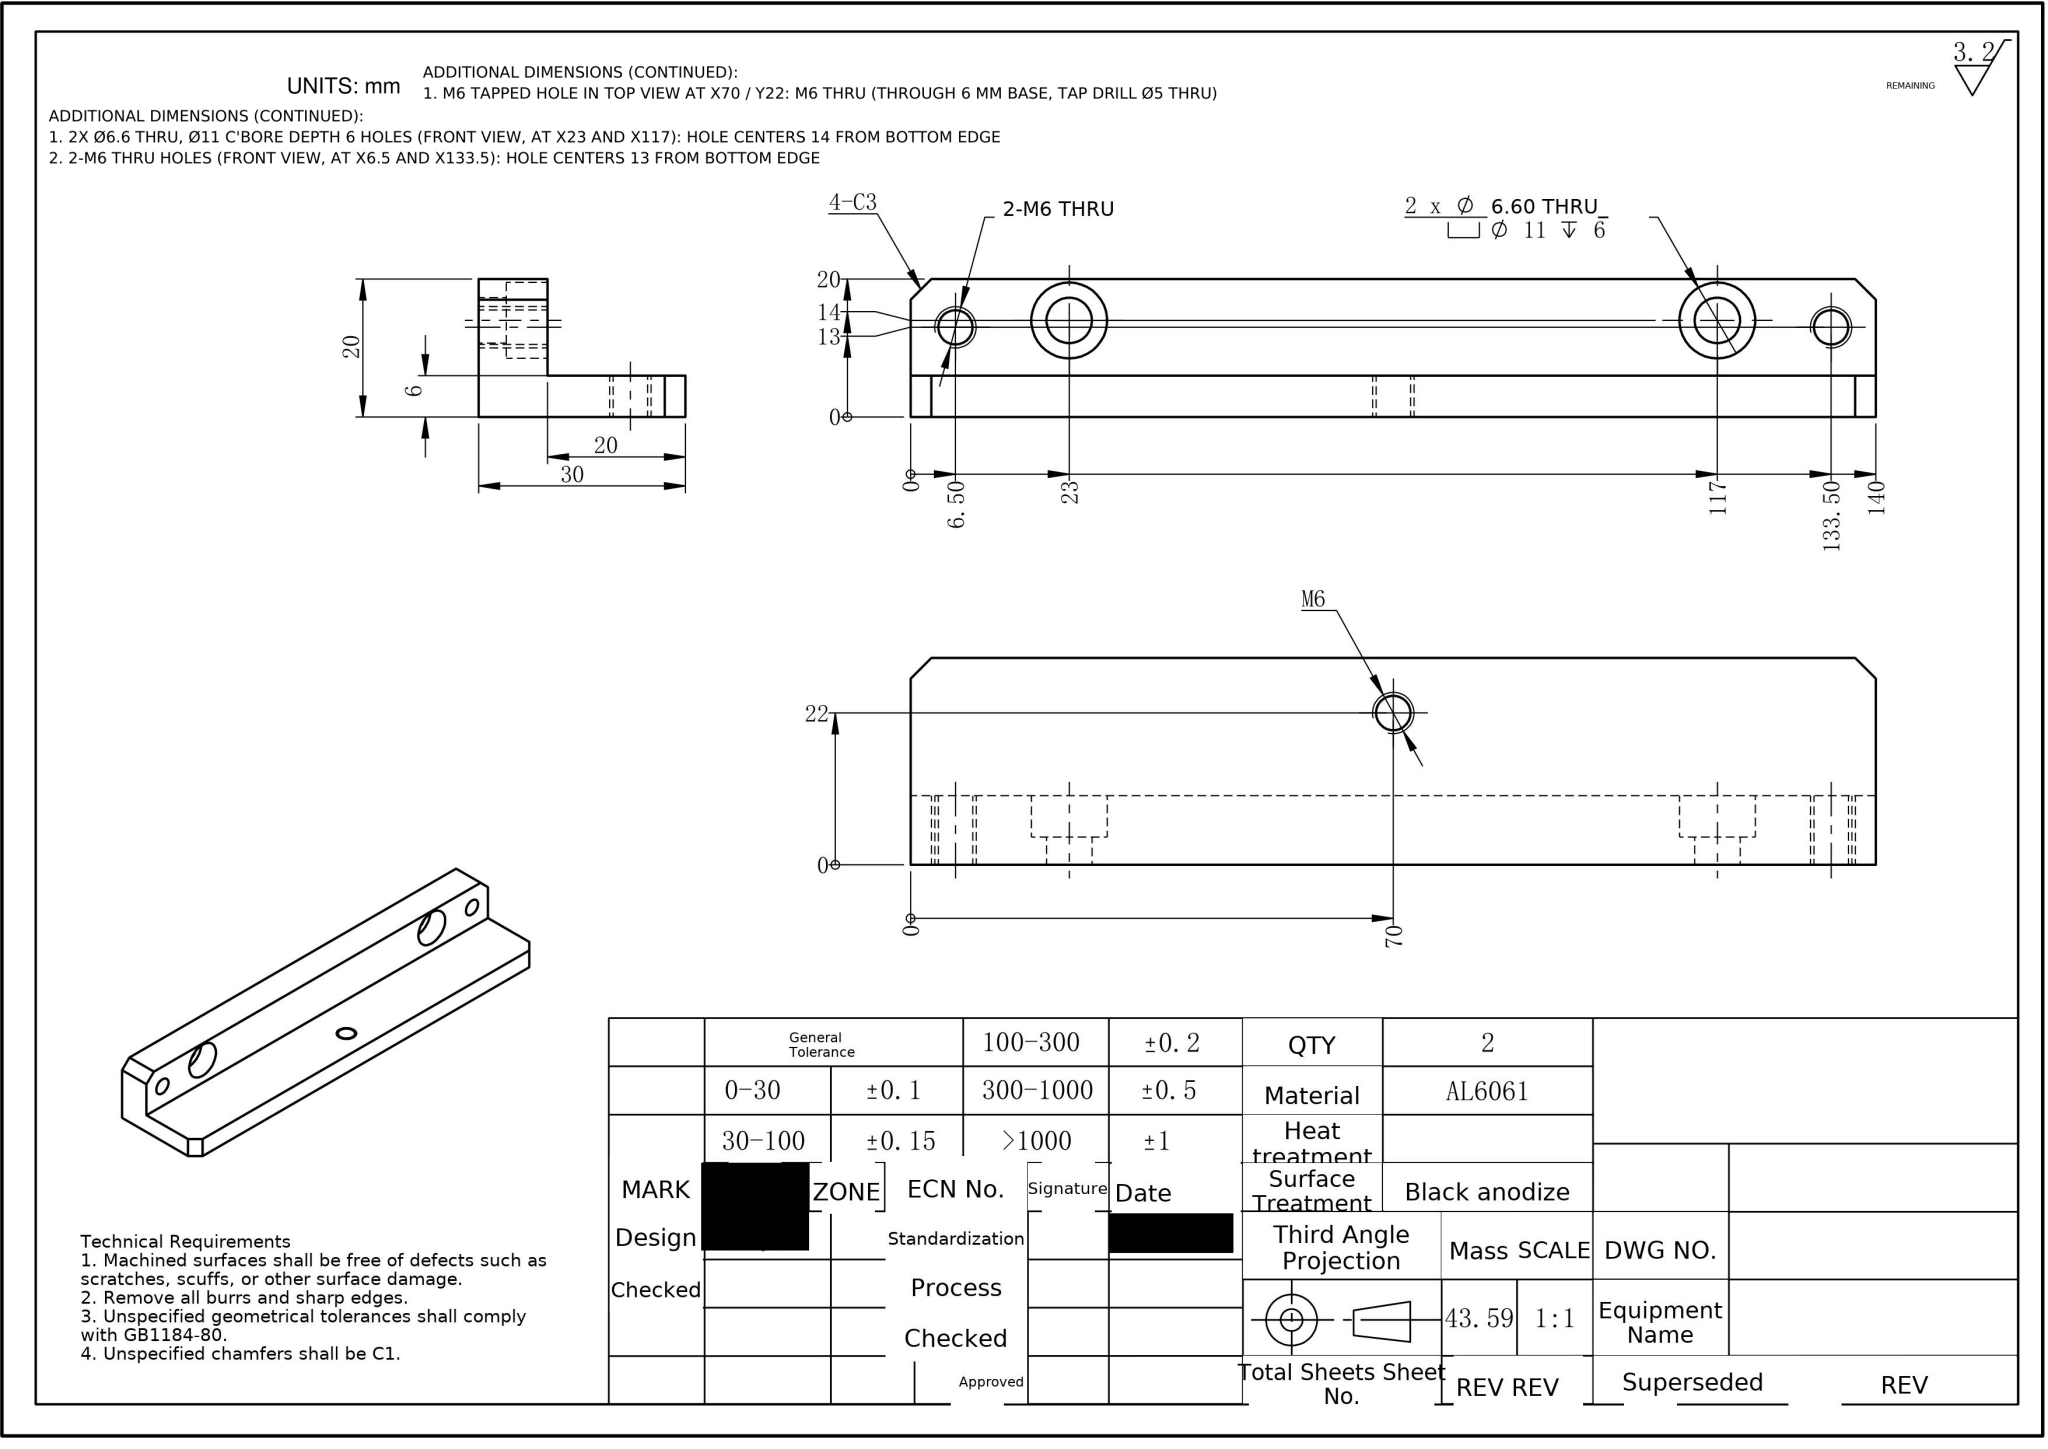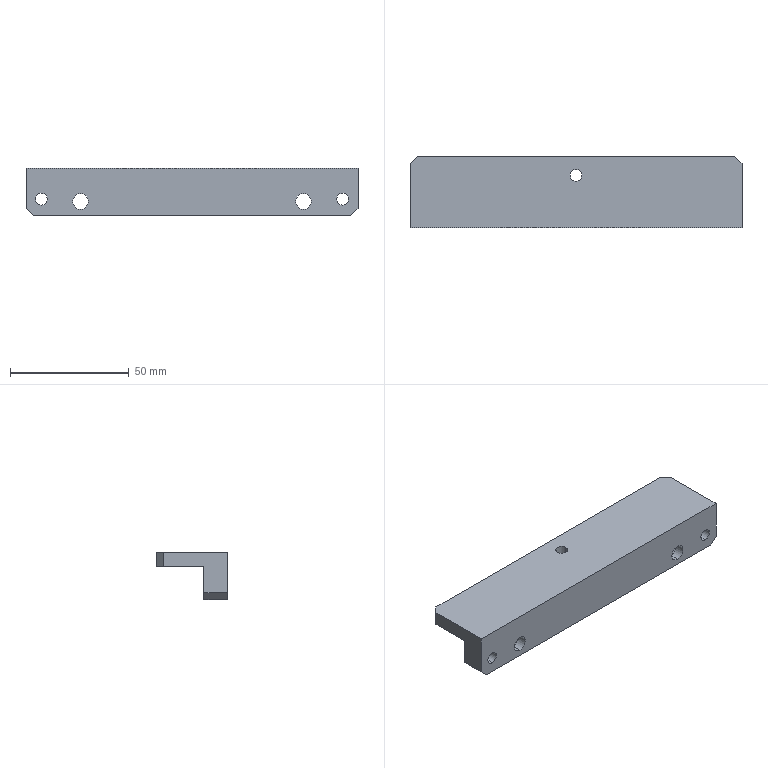Part | NX | mm | 1 solid | 28 faces | box 140 x 30 x 20 mm | volume 42731 mm3 | cylinder 14 | plane 14 | commonest cylinder face diameters 5 x6 11 x4 6.6 x4
STEP:
#1=COLOUR_RGB('',0.7922,0.8196,0.9333);
#2=FILL_AREA_STYLE_COLOUR('',#1);
#3=FILL_AREA_STYLE('',(#2));
#4=SURFACE_STYLE_FILL_AREA(#3);
#5=SURFACE_SIDE_STYLE('',(#4));
#6=SURFACE_STYLE_USAGE(.BOTH.,#5);
#7=PRESENTATION_STYLE_ASSIGNMENT((#6));
#8=CARTESIAN_POINT('',(2.5,17.,10.));
#9=VERTEX_POINT('',#8);
#10=CARTESIAN_POINT('',(-2.5,17.,10.));
#11=VERTEX_POINT('',#10);
#12=CARTESIAN_POINT('',(-0.,17.,10.));
#13=DIRECTION('',(0.,0.,-1.));
#14=DIRECTION('',(-1.,0.,0.));
#15=AXIS2_PLACEMENT_3D('',#12,#13,#14);
#16=CIRCLE('',#15,2.5);
#17=EDGE_CURVE('',#9,#11,#16,.T.);
#18=ORIENTED_EDGE('',*,*,#17,.F.);
#19=CARTESIAN_POINT('',(2.5,17.,4.));
#20=VERTEX_POINT('',#19);
#21=CARTESIAN_POINT('',(2.5,17.,4.));
#22=DIRECTION('',(0.,0.,-1.));
#23=VECTOR('',#22,1000.);
#24=LINE('',#21,#23);
#25=EDGE_CURVE('',#9,#20,#24,.T.);
#26=ORIENTED_EDGE('',*,*,#25,.T.);
#27=CARTESIAN_POINT('',(-2.5,17.,4.));
#28=VERTEX_POINT('',#27);
#29=CARTESIAN_POINT('',(-0.,17.,4.));
#30=DIRECTION('',(0.,0.,-1.));
#31=DIRECTION('',(-1.,0.,0.));
#32=AXIS2_PLACEMENT_3D('',#29,#30,#31);
#33=CIRCLE('',#32,2.5);
#34=EDGE_CURVE('',#20,#28,#33,.T.);
#35=ORIENTED_EDGE('',*,*,#34,.T.);
#36=CARTESIAN_POINT('',(-2.5,17.,4.));
#37=DIRECTION('',(0.,0.,-1.));
#38=VECTOR('',#37,1000.);
#39=LINE('',#36,#38);
#40=EDGE_CURVE('',#11,#28,#39,.T.);
#41=ORIENTED_EDGE('',*,*,#40,.F.);
#42=EDGE_LOOP('',(#18,#26,#35,#41));
#43=FACE_OUTER_BOUND('',#42,.T.);
#44=CARTESIAN_POINT('',(-0.,17.,4.));
#45=DIRECTION('',(0.,0.,-1.));
#46=DIRECTION('',(-1.,0.,0.));
#47=AXIS2_PLACEMENT_3D('',#44,#45,#46);
#48=CYLINDRICAL_SURFACE('',#47,2.5);
#49=ADVANCED_FACE('',(#43),#48,.F.);
#50=CARTESIAN_POINT('',(-63.5,5.,-0.5));
#51=VERTEX_POINT('',#50);
#52=CARTESIAN_POINT('',(-63.5,5.,-5.5));
#53=VERTEX_POINT('',#52);
#54=CARTESIAN_POINT('',(-63.5,5.,-3.));
#55=DIRECTION('',(0.,-1.,0.));
#56=DIRECTION('',(0.,0.,-1.));
#57=AXIS2_PLACEMENT_3D('',#54,#55,#56);
#58=CIRCLE('',#57,2.5);
#59=EDGE_CURVE('',#51,#53,#58,.T.);
#60=ORIENTED_EDGE('',*,*,#59,.F.);
#61=CARTESIAN_POINT('',(-63.5,-5.,-0.5));
#62=VERTEX_POINT('',#61);
#63=CARTESIAN_POINT('',(-63.5,-5.,-0.5));
#64=DIRECTION('',(0.,-1.,0.));
#65=VECTOR('',#64,1000.);
#66=LINE('',#63,#65);
#67=EDGE_CURVE('',#51,#62,#66,.T.);
#68=ORIENTED_EDGE('',*,*,#67,.T.);
#69=CARTESIAN_POINT('',(-63.5,-5.,-5.5));
#70=VERTEX_POINT('',#69);
#71=CARTESIAN_POINT('',(-63.5,-5.,-3.));
#72=DIRECTION('',(0.,-1.,0.));
#73=DIRECTION('',(0.,0.,-1.));
#74=AXIS2_PLACEMENT_3D('',#71,#72,#73);
#75=CIRCLE('',#74,2.5);
#76=EDGE_CURVE('',#62,#70,#75,.T.);
#77=ORIENTED_EDGE('',*,*,#76,.T.);
#78=CARTESIAN_POINT('',(-63.5,-5.,-5.5));
#79=DIRECTION('',(0.,-1.,0.));
#80=VECTOR('',#79,1000.);
#81=LINE('',#78,#80);
#82=EDGE_CURVE('',#53,#70,#81,.T.);
#83=ORIENTED_EDGE('',*,*,#82,.F.);
#84=EDGE_LOOP('',(#60,#68,#77,#83));
#85=FACE_OUTER_BOUND('',#84,.T.);
#86=CARTESIAN_POINT('',(-63.5,-5.,-3.));
#87=DIRECTION('',(0.,-1.,0.));
#88=DIRECTION('',(0.,0.,-1.));
#89=AXIS2_PLACEMENT_3D('',#86,#87,#88);
#90=CYLINDRICAL_SURFACE('',#89,2.5);
#91=ADVANCED_FACE('',(#85),#90,.F.);
#92=CARTESIAN_POINT('',(63.5,5.,-0.5));
#93=VERTEX_POINT('',#92);
#94=CARTESIAN_POINT('',(63.5,5.,-5.5));
#95=VERTEX_POINT('',#94);
#96=CARTESIAN_POINT('',(63.5,5.,-3.));
#97=DIRECTION('',(0.,-1.,0.));
#98=DIRECTION('',(0.,0.,-1.));
#99=AXIS2_PLACEMENT_3D('',#96,#97,#98);
#100=CIRCLE('',#99,2.5);
#101=EDGE_CURVE('',#93,#95,#100,.T.);
#102=ORIENTED_EDGE('',*,*,#101,.F.);
#103=CARTESIAN_POINT('',(63.5,-5.,-0.5));
#104=VERTEX_POINT('',#103);
#105=CARTESIAN_POINT('',(63.5,-5.,-0.5));
#106=DIRECTION('',(0.,-1.,0.));
#107=VECTOR('',#106,1000.);
#108=LINE('',#105,#107);
#109=EDGE_CURVE('',#93,#104,#108,.T.);
#110=ORIENTED_EDGE('',*,*,#109,.T.);
#111=CARTESIAN_POINT('',(63.5,-5.,-5.5));
#112=VERTEX_POINT('',#111);
#113=CARTESIAN_POINT('',(63.5,-5.,-3.));
#114=DIRECTION('',(0.,-1.,0.));
#115=DIRECTION('',(0.,0.,-1.));
#116=AXIS2_PLACEMENT_3D('',#113,#114,#115);
#117=CIRCLE('',#116,2.5);
#118=EDGE_CURVE('',#104,#112,#117,.T.);
#119=ORIENTED_EDGE('',*,*,#118,.T.);
#120=CARTESIAN_POINT('',(63.5,-5.,-5.5));
#121=DIRECTION('',(0.,-1.,0.));
#122=VECTOR('',#121,1000.);
#123=LINE('',#120,#122);
#124=EDGE_CURVE('',#95,#112,#123,.T.);
#125=ORIENTED_EDGE('',*,*,#124,.F.);
#126=EDGE_LOOP('',(#102,#110,#119,#125));
#127=FACE_OUTER_BOUND('',#126,.T.);
#128=CARTESIAN_POINT('',(63.5,-5.,-3.));
#129=DIRECTION('',(0.,-1.,0.));
#130=DIRECTION('',(0.,0.,-1.));
#131=AXIS2_PLACEMENT_3D('',#128,#129,#130);
#132=CYLINDRICAL_SURFACE('',#131,2.5);
#133=ADVANCED_FACE('',(#127),#132,.F.);
#134=CARTESIAN_POINT('',(-47.,-1.,-9.5));
#135=VERTEX_POINT('',#134);
#136=CARTESIAN_POINT('',(-47.,-1.,1.5));
#137=VERTEX_POINT('',#136);
#138=CARTESIAN_POINT('',(-47.,-1.,-4.));
#139=DIRECTION('',(0.,1.,0.));
#140=DIRECTION('',(0.,0.,1.));
#141=AXIS2_PLACEMENT_3D('',#138,#139,#140);
#142=CIRCLE('',#141,5.5);
#143=EDGE_CURVE('',#135,#137,#142,.T.);
#144=ORIENTED_EDGE('',*,*,#143,.F.);
#145=CARTESIAN_POINT('',(-47.,5.,-9.5));
#146=VERTEX_POINT('',#145);
#147=CARTESIAN_POINT('',(-47.,5.,-9.5));
#148=DIRECTION('',(0.,1.,0.));
#149=VECTOR('',#148,1000.);
#150=LINE('',#147,#149);
#151=EDGE_CURVE('',#135,#146,#150,.T.);
#152=ORIENTED_EDGE('',*,*,#151,.T.);
#153=CARTESIAN_POINT('',(-47.,5.,1.5));
#154=VERTEX_POINT('',#153);
#155=CARTESIAN_POINT('',(-47.,5.,-4.));
#156=DIRECTION('',(0.,1.,0.));
#157=DIRECTION('',(0.,0.,1.));
#158=AXIS2_PLACEMENT_3D('',#155,#156,#157);
#159=CIRCLE('',#158,5.5);
#160=EDGE_CURVE('',#146,#154,#159,.T.);
#161=ORIENTED_EDGE('',*,*,#160,.T.);
#162=CARTESIAN_POINT('',(-47.,5.,1.5));
#163=DIRECTION('',(0.,1.,0.));
#164=VECTOR('',#163,1000.);
#165=LINE('',#162,#164);
#166=EDGE_CURVE('',#137,#154,#165,.T.);
#167=ORIENTED_EDGE('',*,*,#166,.F.);
#168=EDGE_LOOP('',(#144,#152,#161,#167));
#169=FACE_OUTER_BOUND('',#168,.T.);
#170=CARTESIAN_POINT('',(-47.,5.,-4.));
#171=DIRECTION('',(0.,1.,0.));
#172=DIRECTION('',(0.,0.,1.));
#173=AXIS2_PLACEMENT_3D('',#170,#171,#172);
#174=CYLINDRICAL_SURFACE('',#173,5.5);
#175=ADVANCED_FACE('',(#169),#174,.F.);
#176=CARTESIAN_POINT('',(-47.,-5.,-7.3));
#177=VERTEX_POINT('',#176);
#178=CARTESIAN_POINT('',(-47.,-5.,-0.7));
#179=VERTEX_POINT('',#178);
#180=CARTESIAN_POINT('',(-47.,-5.,-4.));
#181=DIRECTION('',(0.,1.,0.));
#182=DIRECTION('',(0.,0.,1.));
#183=AXIS2_PLACEMENT_3D('',#180,#181,#182);
#184=CIRCLE('',#183,3.3);
#185=EDGE_CURVE('',#177,#179,#184,.T.);
#186=ORIENTED_EDGE('',*,*,#185,.F.);
#187=CARTESIAN_POINT('',(-47.,-1.,-7.3));
#188=VERTEX_POINT('',#187);
#189=CARTESIAN_POINT('',(-47.,5.,-7.3));
#190=DIRECTION('',(0.,1.,0.));
#191=VECTOR('',#190,1000.);
#192=LINE('',#189,#191);
#193=EDGE_CURVE('',#177,#188,#192,.T.);
#194=ORIENTED_EDGE('',*,*,#193,.T.);
#195=CARTESIAN_POINT('',(-47.,-1.,-0.7));
#196=VERTEX_POINT('',#195);
#197=CARTESIAN_POINT('',(-47.,-1.,-4.));
#198=DIRECTION('',(0.,1.,0.));
#199=DIRECTION('',(0.,0.,1.));
#200=AXIS2_PLACEMENT_3D('',#197,#198,#199);
#201=CIRCLE('',#200,3.3);
#202=EDGE_CURVE('',#188,#196,#201,.T.);
#203=ORIENTED_EDGE('',*,*,#202,.T.);
#204=CARTESIAN_POINT('',(-47.,5.,-0.7));
#205=DIRECTION('',(0.,1.,0.));
#206=VECTOR('',#205,1000.);
#207=LINE('',#204,#206);
#208=EDGE_CURVE('',#179,#196,#207,.T.);
#209=ORIENTED_EDGE('',*,*,#208,.F.);
#210=EDGE_LOOP('',(#186,#194,#203,#209));
#211=FACE_OUTER_BOUND('',#210,.T.);
#212=CARTESIAN_POINT('',(-47.,5.,-4.));
#213=DIRECTION('',(0.,1.,0.));
#214=DIRECTION('',(0.,0.,1.));
#215=AXIS2_PLACEMENT_3D('',#212,#213,#214);
#216=CYLINDRICAL_SURFACE('',#215,3.3);
#217=ADVANCED_FACE('',(#211),#216,.F.);
#218=CARTESIAN_POINT('',(47.,-1.,-9.5));
#219=VERTEX_POINT('',#218);
#220=CARTESIAN_POINT('',(47.,-1.,1.5));
#221=VERTEX_POINT('',#220);
#222=CARTESIAN_POINT('',(47.,-1.,-4.));
#223=DIRECTION('',(0.,1.,0.));
#224=DIRECTION('',(0.,0.,1.));
#225=AXIS2_PLACEMENT_3D('',#222,#223,#224);
#226=CIRCLE('',#225,5.5);
#227=EDGE_CURVE('',#219,#221,#226,.T.);
#228=ORIENTED_EDGE('',*,*,#227,.F.);
#229=CARTESIAN_POINT('',(47.,5.,-9.5));
#230=VERTEX_POINT('',#229);
#231=CARTESIAN_POINT('',(47.,5.,-9.5));
#232=DIRECTION('',(0.,1.,0.));
#233=VECTOR('',#232,1000.);
#234=LINE('',#231,#233);
#235=EDGE_CURVE('',#219,#230,#234,.T.);
#236=ORIENTED_EDGE('',*,*,#235,.T.);
#237=CARTESIAN_POINT('',(47.,5.,1.5));
#238=VERTEX_POINT('',#237);
#239=CARTESIAN_POINT('',(47.,5.,-4.));
#240=DIRECTION('',(0.,1.,0.));
#241=DIRECTION('',(0.,0.,1.));
#242=AXIS2_PLACEMENT_3D('',#239,#240,#241);
#243=CIRCLE('',#242,5.5);
#244=EDGE_CURVE('',#230,#238,#243,.T.);
#245=ORIENTED_EDGE('',*,*,#244,.T.);
#246=CARTESIAN_POINT('',(47.,5.,1.5));
#247=DIRECTION('',(0.,1.,0.));
#248=VECTOR('',#247,1000.);
#249=LINE('',#246,#248);
#250=EDGE_CURVE('',#221,#238,#249,.T.);
#251=ORIENTED_EDGE('',*,*,#250,.F.);
#252=EDGE_LOOP('',(#228,#236,#245,#251));
#253=FACE_OUTER_BOUND('',#252,.T.);
#254=CARTESIAN_POINT('',(47.,5.,-4.));
#255=DIRECTION('',(0.,1.,0.));
#256=DIRECTION('',(0.,0.,1.));
#257=AXIS2_PLACEMENT_3D('',#254,#255,#256);
#258=CYLINDRICAL_SURFACE('',#257,5.5);
#259=ADVANCED_FACE('',(#253),#258,.F.);
#260=CARTESIAN_POINT('',(47.,-5.,-7.3));
#261=VERTEX_POINT('',#260);
#262=CARTESIAN_POINT('',(47.,-5.,-0.7));
#263=VERTEX_POINT('',#262);
#264=CARTESIAN_POINT('',(47.,-5.,-4.));
#265=DIRECTION('',(0.,1.,0.));
#266=DIRECTION('',(0.,0.,1.));
#267=AXIS2_PLACEMENT_3D('',#264,#265,#266);
#268=CIRCLE('',#267,3.3);
#269=EDGE_CURVE('',#261,#263,#268,.T.);
#270=ORIENTED_EDGE('',*,*,#269,.F.);
#271=CARTESIAN_POINT('',(47.,-1.,-7.3));
#272=VERTEX_POINT('',#271);
#273=CARTESIAN_POINT('',(47.,5.,-7.3));
#274=DIRECTION('',(0.,1.,0.));
#275=VECTOR('',#274,1000.);
#276=LINE('',#273,#275);
#277=EDGE_CURVE('',#261,#272,#276,.T.);
#278=ORIENTED_EDGE('',*,*,#277,.T.);
#279=CARTESIAN_POINT('',(47.,-1.,-0.7));
#280=VERTEX_POINT('',#279);
#281=CARTESIAN_POINT('',(47.,-1.,-4.));
#282=DIRECTION('',(0.,1.,0.));
#283=DIRECTION('',(0.,0.,1.));
#284=AXIS2_PLACEMENT_3D('',#281,#282,#283);
#285=CIRCLE('',#284,3.3);
#286=EDGE_CURVE('',#272,#280,#285,.T.);
#287=ORIENTED_EDGE('',*,*,#286,.T.);
#288=CARTESIAN_POINT('',(47.,5.,-0.7));
#289=DIRECTION('',(0.,1.,0.));
#290=VECTOR('',#289,1000.);
#291=LINE('',#288,#290);
#292=EDGE_CURVE('',#263,#280,#291,.T.);
#293=ORIENTED_EDGE('',*,*,#292,.F.);
#294=EDGE_LOOP('',(#270,#278,#287,#293));
#295=FACE_OUTER_BOUND('',#294,.T.);
#296=CARTESIAN_POINT('',(47.,5.,-4.));
#297=DIRECTION('',(0.,1.,0.));
#298=DIRECTION('',(0.,0.,1.));
#299=AXIS2_PLACEMENT_3D('',#296,#297,#298);
#300=CYLINDRICAL_SURFACE('',#299,3.3);
#301=ADVANCED_FACE('',(#295),#300,.F.);
#302=CARTESIAN_POINT('',(-63.5,5.,-3.));
#303=DIRECTION('',(0.,-1.,0.));
#304=DIRECTION('',(0.,0.,-1.));
#305=AXIS2_PLACEMENT_3D('',#302,#303,#304);
#306=CIRCLE('',#305,2.5);
#307=EDGE_CURVE('',#53,#51,#306,.T.);
#308=ORIENTED_EDGE('',*,*,#307,.T.);
#309=ORIENTED_EDGE('',*,*,#59,.T.);
#310=EDGE_LOOP('',(#308,#309));
#311=FACE_BOUND('',#310,.T.);
#312=CARTESIAN_POINT('',(63.5,5.,-3.));
#313=DIRECTION('',(0.,-1.,0.));
#314=DIRECTION('',(0.,0.,-1.));
#315=AXIS2_PLACEMENT_3D('',#312,#313,#314);
#316=CIRCLE('',#315,2.5);
#317=EDGE_CURVE('',#95,#93,#316,.T.);
#318=ORIENTED_EDGE('',*,*,#317,.T.);
#319=ORIENTED_EDGE('',*,*,#101,.T.);
#320=EDGE_LOOP('',(#318,#319));
#321=FACE_BOUND('',#320,.T.);
#322=CARTESIAN_POINT('',(47.,5.,-4.));
#323=DIRECTION('',(0.,1.,0.));
#324=DIRECTION('',(0.,0.,1.));
#325=AXIS2_PLACEMENT_3D('',#322,#323,#324);
#326=CIRCLE('',#325,5.5);
#327=EDGE_CURVE('',#238,#230,#326,.T.);
#328=ORIENTED_EDGE('',*,*,#327,.F.);
#329=ORIENTED_EDGE('',*,*,#244,.F.);
#330=EDGE_LOOP('',(#328,#329));
#331=FACE_BOUND('',#330,.T.);
#332=CARTESIAN_POINT('',(-47.,5.,-4.));
#333=DIRECTION('',(0.,1.,0.));
#334=DIRECTION('',(0.,0.,1.));
#335=AXIS2_PLACEMENT_3D('',#332,#333,#334);
#336=CIRCLE('',#335,5.5);
#337=EDGE_CURVE('',#154,#146,#336,.T.);
#338=ORIENTED_EDGE('',*,*,#337,.F.);
#339=ORIENTED_EDGE('',*,*,#160,.F.);
#340=EDGE_LOOP('',(#338,#339));
#341=FACE_BOUND('',#340,.T.);
#342=CARTESIAN_POINT('',(70.,5.,4.));
#343=VERTEX_POINT('',#342);
#344=CARTESIAN_POINT('',(70.,5.,-7.));
#345=VERTEX_POINT('',#344);
#346=CARTESIAN_POINT('',(70.,5.,10.));
#347=DIRECTION('',(0.,0.,-1.));
#348=VECTOR('',#347,1000.);
#349=LINE('',#346,#348);
#350=EDGE_CURVE('',#343,#345,#349,.T.);
#351=ORIENTED_EDGE('',*,*,#350,.T.);
#352=CARTESIAN_POINT('',(67.,5.,-10.));
#353=VERTEX_POINT('',#352);
#354=CARTESIAN_POINT('',(67.,5.,-10.));
#355=DIRECTION('',(-0.7071,0.,-0.7071));
#356=VECTOR('',#355,1000.);
#357=LINE('',#354,#356);
#358=EDGE_CURVE('',#345,#353,#357,.T.);
#359=ORIENTED_EDGE('',*,*,#358,.T.);
#360=CARTESIAN_POINT('',(-67.,5.,-10.));
#361=VERTEX_POINT('',#360);
#362=CARTESIAN_POINT('',(-70.,5.,-10.));
#363=DIRECTION('',(-1.,0.,0.));
#364=VECTOR('',#363,1000.);
#365=LINE('',#362,#364);
#366=EDGE_CURVE('',#353,#361,#365,.T.);
#367=ORIENTED_EDGE('',*,*,#366,.T.);
#368=CARTESIAN_POINT('',(-70.,5.,-7.));
#369=VERTEX_POINT('',#368);
#370=CARTESIAN_POINT('',(-70.,5.,-7.));
#371=DIRECTION('',(-0.7071,0.,0.7071));
#372=VECTOR('',#371,1000.);
#373=LINE('',#370,#372);
#374=EDGE_CURVE('',#361,#369,#373,.T.);
#375=ORIENTED_EDGE('',*,*,#374,.T.);
#376=CARTESIAN_POINT('',(-70.,5.,4.));
#377=VERTEX_POINT('',#376);
#378=CARTESIAN_POINT('',(-70.,5.,10.));
#379=DIRECTION('',(0.,0.,1.));
#380=VECTOR('',#379,1000.);
#381=LINE('',#378,#380);
#382=EDGE_CURVE('',#369,#377,#381,.T.);
#383=ORIENTED_EDGE('',*,*,#382,.T.);
#384=CARTESIAN_POINT('',(-70.,5.,4.));
#385=DIRECTION('',(-1.,0.,0.));
#386=VECTOR('',#385,1000.);
#387=LINE('',#384,#386);
#388=EDGE_CURVE('',#343,#377,#387,.T.);
#389=ORIENTED_EDGE('',*,*,#388,.F.);
#390=EDGE_LOOP('',(#351,#359,#367,#375,#383,#389));
#391=FACE_OUTER_BOUND('',#390,.T.);
#392=CARTESIAN_POINT('',(0.,5.,0.));
#393=DIRECTION('',(0.,-1.,0.));
#394=DIRECTION('',(0.,0.,-1.));
#395=AXIS2_PLACEMENT_3D('',#392,#393,#394);
#396=PLANE('',#395);
#397=ADVANCED_FACE('',(#311,#321,#331,#341,#391),#396,.F.);
#398=CARTESIAN_POINT('',(70.,-5.,10.));
#399=VERTEX_POINT('',#398);
#400=CARTESIAN_POINT('',(70.,-5.,-7.));
#401=VERTEX_POINT('',#400);
#402=CARTESIAN_POINT('',(70.,-5.,10.));
#403=DIRECTION('',(0.,0.,-1.));
#404=VECTOR('',#403,1000.);
#405=LINE('',#402,#404);
#406=EDGE_CURVE('',#399,#401,#405,.T.);
#407=ORIENTED_EDGE('',*,*,#406,.T.);
#408=CARTESIAN_POINT('',(70.,5.,-7.));
#409=DIRECTION('',(0.,1.,0.));
#410=VECTOR('',#409,1000.);
#411=LINE('',#408,#410);
#412=EDGE_CURVE('',#401,#345,#411,.T.);
#413=ORIENTED_EDGE('',*,*,#412,.T.);
#414=ORIENTED_EDGE('',*,*,#350,.F.);
#415=CARTESIAN_POINT('',(70.,22.,4.));
#416=VERTEX_POINT('',#415);
#417=CARTESIAN_POINT('',(70.,25.,4.));
#418=DIRECTION('',(0.,-1.,0.));
#419=VECTOR('',#418,1000.);
#420=LINE('',#417,#419);
#421=EDGE_CURVE('',#416,#343,#420,.T.);
#422=ORIENTED_EDGE('',*,*,#421,.F.);
#423=CARTESIAN_POINT('',(70.,22.,10.));
#424=VERTEX_POINT('',#423);
#425=CARTESIAN_POINT('',(70.,22.,10.));
#426=DIRECTION('',(0.,0.,1.));
#427=VECTOR('',#426,1000.);
#428=LINE('',#425,#427);
#429=EDGE_CURVE('',#416,#424,#428,.T.);
#430=ORIENTED_EDGE('',*,*,#429,.T.);
#431=CARTESIAN_POINT('',(70.,5.,10.));
#432=DIRECTION('',(0.,-1.,0.));
#433=VECTOR('',#432,1000.);
#434=LINE('',#431,#433);
#435=EDGE_CURVE('',#424,#399,#434,.T.);
#436=ORIENTED_EDGE('',*,*,#435,.T.);
#437=EDGE_LOOP('',(#407,#413,#414,#422,#430,#436));
#438=FACE_OUTER_BOUND('',#437,.T.);
#439=CARTESIAN_POINT('',(70.,5.,10.));
#440=DIRECTION('',(-1.,0.,0.));
#441=DIRECTION('',(0.,0.,1.));
#442=AXIS2_PLACEMENT_3D('',#439,#440,#441);
#443=PLANE('',#442);
#444=ADVANCED_FACE('',(#438),#443,.F.);
#445=ORIENTED_EDGE('',*,*,#366,.F.);
#446=CARTESIAN_POINT('',(67.,-5.,-10.));
#447=VERTEX_POINT('',#446);
#448=CARTESIAN_POINT('',(67.,5.,-10.));
#449=DIRECTION('',(0.,-1.,0.));
#450=VECTOR('',#449,1000.);
#451=LINE('',#448,#450);
#452=EDGE_CURVE('',#353,#447,#451,.T.);
#453=ORIENTED_EDGE('',*,*,#452,.T.);
#454=CARTESIAN_POINT('',(-67.,-5.,-10.));
#455=VERTEX_POINT('',#454);
#456=CARTESIAN_POINT('',(-70.,-5.,-10.));
#457=DIRECTION('',(-1.,0.,0.));
#458=VECTOR('',#457,1000.);
#459=LINE('',#456,#458);
#460=EDGE_CURVE('',#447,#455,#459,.T.);
#461=ORIENTED_EDGE('',*,*,#460,.T.);
#462=CARTESIAN_POINT('',(-67.,5.,-10.));
#463=DIRECTION('',(0.,1.,0.));
#464=VECTOR('',#463,1000.);
#465=LINE('',#462,#464);
#466=EDGE_CURVE('',#455,#361,#465,.T.);
#467=ORIENTED_EDGE('',*,*,#466,.T.);
#468=EDGE_LOOP('',(#445,#453,#461,#467));
#469=FACE_OUTER_BOUND('',#468,.T.);
#470=CARTESIAN_POINT('',(-70.,5.,-10.));
#471=DIRECTION('',(0.,0.,1.));
#472=DIRECTION('',(1.,0.,0.));
#473=AXIS2_PLACEMENT_3D('',#470,#471,#472);
#474=PLANE('',#473);
#475=ADVANCED_FACE('',(#469),#474,.F.);
#476=ORIENTED_EDGE('',*,*,#382,.F.);
#477=CARTESIAN_POINT('',(-70.,-5.,-7.));
#478=VERTEX_POINT('',#477);
#479=CARTESIAN_POINT('',(-70.,5.,-7.));
#480=DIRECTION('',(0.,-1.,0.));
#481=VECTOR('',#480,1000.);
#482=LINE('',#479,#481);
#483=EDGE_CURVE('',#369,#478,#482,.T.);
#484=ORIENTED_EDGE('',*,*,#483,.T.);
#485=CARTESIAN_POINT('',(-70.,-5.,10.));
#486=VERTEX_POINT('',#485);
#487=CARTESIAN_POINT('',(-70.,-5.,10.));
#488=DIRECTION('',(0.,0.,1.));
#489=VECTOR('',#488,1000.);
#490=LINE('',#487,#489);
#491=EDGE_CURVE('',#478,#486,#490,.T.);
#492=ORIENTED_EDGE('',*,*,#491,.T.);
#493=CARTESIAN_POINT('',(-70.,22.,10.));
#494=VERTEX_POINT('',#493);
#495=CARTESIAN_POINT('',(-70.,5.,10.));
#496=DIRECTION('',(0.,-1.,0.));
#497=VECTOR('',#496,1000.);
#498=LINE('',#495,#497);
#499=EDGE_CURVE('',#494,#486,#498,.T.);
#500=ORIENTED_EDGE('',*,*,#499,.F.);
#501=CARTESIAN_POINT('',(-70.,22.,4.));
#502=VERTEX_POINT('',#501);
#503=CARTESIAN_POINT('',(-70.,22.,10.));
#504=DIRECTION('',(0.,0.,-1.));
#505=VECTOR('',#504,1000.);
#506=LINE('',#503,#505);
#507=EDGE_CURVE('',#494,#502,#506,.T.);
#508=ORIENTED_EDGE('',*,*,#507,.T.);
#509=CARTESIAN_POINT('',(-70.,25.,4.));
#510=DIRECTION('',(0.,-1.,0.));
#511=VECTOR('',#510,1000.);
#512=LINE('',#509,#511);
#513=EDGE_CURVE('',#502,#377,#512,.T.);
#514=ORIENTED_EDGE('',*,*,#513,.T.);
#515=EDGE_LOOP('',(#476,#484,#492,#500,#508,#514));
#516=FACE_OUTER_BOUND('',#515,.T.);
#517=CARTESIAN_POINT('',(-70.,5.,10.));
#518=DIRECTION('',(1.,0.,0.));
#519=DIRECTION('',(0.,0.,-1.));
#520=AXIS2_PLACEMENT_3D('',#517,#518,#519);
#521=PLANE('',#520);
#522=ADVANCED_FACE('',(#516),#521,.F.);
#523=CARTESIAN_POINT('',(-0.,17.,10.));
#524=DIRECTION('',(0.,0.,-1.));
#525=DIRECTION('',(-1.,0.,0.));
#526=AXIS2_PLACEMENT_3D('',#523,#524,#525);
#527=CIRCLE('',#526,2.5);
#528=EDGE_CURVE('',#11,#9,#527,.T.);
#529=ORIENTED_EDGE('',*,*,#528,.T.);
#530=ORIENTED_EDGE('',*,*,#17,.T.);
#531=EDGE_LOOP('',(#529,#530));
#532=FACE_BOUND('',#531,.T.);
#533=CARTESIAN_POINT('',(-67.,25.,10.));
#534=VERTEX_POINT('',#533);
#535=CARTESIAN_POINT('',(67.,25.,10.));
#536=VERTEX_POINT('',#535);
#537=CARTESIAN_POINT('',(-70.,25.,10.));
#538=DIRECTION('',(1.,0.,0.));
#539=VECTOR('',#538,1000.);
#540=LINE('',#537,#539);
#541=EDGE_CURVE('',#534,#536,#540,.T.);
#542=ORIENTED_EDGE('',*,*,#541,.F.);
#543=CARTESIAN_POINT('',(-67.,25.,10.));
#544=DIRECTION('',(-0.7071,-0.7071,0.));
#545=VECTOR('',#544,1000.);
#546=LINE('',#543,#545);
#547=EDGE_CURVE('',#534,#494,#546,.T.);
#548=ORIENTED_EDGE('',*,*,#547,.T.);
#549=ORIENTED_EDGE('',*,*,#499,.T.);
#550=CARTESIAN_POINT('',(-70.,-5.,10.));
#551=DIRECTION('',(1.,0.,0.));
#552=VECTOR('',#551,1000.);
#553=LINE('',#550,#552);
#554=EDGE_CURVE('',#486,#399,#553,.T.);
#555=ORIENTED_EDGE('',*,*,#554,.T.);
#556=ORIENTED_EDGE('',*,*,#435,.F.);
#557=CARTESIAN_POINT('',(67.,25.,10.));
#558=DIRECTION('',(-0.7071,0.7071,0.));
#559=VECTOR('',#558,1000.);
#560=LINE('',#557,#559);
#561=EDGE_CURVE('',#424,#536,#560,.T.);
#562=ORIENTED_EDGE('',*,*,#561,.T.);
#563=EDGE_LOOP('',(#542,#548,#549,#555,#556,#562));
#564=FACE_OUTER_BOUND('',#563,.T.);
#565=CARTESIAN_POINT('',(-70.,5.,10.));
#566=DIRECTION('',(0.,0.,-1.));
#567=DIRECTION('',(-1.,0.,0.));
#568=AXIS2_PLACEMENT_3D('',#565,#566,#567);
#569=PLANE('',#568);
#570=ADVANCED_FACE('',(#532,#564),#569,.F.);
#571=CARTESIAN_POINT('',(-63.5,-5.,-3.));
#572=DIRECTION('',(0.,-1.,0.));
#573=DIRECTION('',(0.,0.,-1.));
#574=AXIS2_PLACEMENT_3D('',#571,#572,#573);
#575=CIRCLE('',#574,2.5);
#576=EDGE_CURVE('',#70,#62,#575,.T.);
#577=ORIENTED_EDGE('',*,*,#576,.F.);
#578=ORIENTED_EDGE('',*,*,#76,.F.);
#579=EDGE_LOOP('',(#577,#578));
#580=FACE_BOUND('',#579,.T.);
#581=CARTESIAN_POINT('',(63.5,-5.,-3.));
#582=DIRECTION('',(0.,-1.,0.));
#583=DIRECTION('',(0.,0.,-1.));
#584=AXIS2_PLACEMENT_3D('',#581,#582,#583);
#585=CIRCLE('',#584,2.5);
#586=EDGE_CURVE('',#112,#104,#585,.T.);
#587=ORIENTED_EDGE('',*,*,#586,.F.);
#588=ORIENTED_EDGE('',*,*,#118,.F.);
#589=EDGE_LOOP('',(#587,#588));
#590=FACE_BOUND('',#589,.T.);
#591=CARTESIAN_POINT('',(-47.,-5.,-4.));
#592=DIRECTION('',(0.,1.,0.));
#593=DIRECTION('',(0.,0.,1.));
#594=AXIS2_PLACEMENT_3D('',#591,#592,#593);
#595=CIRCLE('',#594,3.3);
#596=EDGE_CURVE('',#179,#177,#595,.T.);
#597=ORIENTED_EDGE('',*,*,#596,.T.);
#598=ORIENTED_EDGE('',*,*,#185,.T.);
#599=EDGE_LOOP('',(#597,#598));
#600=FACE_BOUND('',#599,.T.);
#601=CARTESIAN_POINT('',(47.,-5.,-4.));
#602=DIRECTION('',(0.,1.,0.));
#603=DIRECTION('',(0.,0.,1.));
#604=AXIS2_PLACEMENT_3D('',#601,#602,#603);
#605=CIRCLE('',#604,3.3);
#606=EDGE_CURVE('',#263,#261,#605,.T.);
#607=ORIENTED_EDGE('',*,*,#606,.T.);
#608=ORIENTED_EDGE('',*,*,#269,.T.);
#609=EDGE_LOOP('',(#607,#608));
#610=FACE_BOUND('',#609,.T.);
#611=ORIENTED_EDGE('',*,*,#460,.F.);
#612=CARTESIAN_POINT('',(38.5,-5.,-38.5));
#613=DIRECTION('',(0.7071,0.,0.7071));
#614=VECTOR('',#613,1000.);
#615=LINE('',#612,#614);
#616=EDGE_CURVE('',#447,#401,#615,.T.);
#617=ORIENTED_EDGE('',*,*,#616,.T.);
#618=ORIENTED_EDGE('',*,*,#406,.F.);
#619=ORIENTED_EDGE('',*,*,#554,.F.);
#620=ORIENTED_EDGE('',*,*,#491,.F.);
#621=CARTESIAN_POINT('',(-38.5,-5.,-38.5));
#622=DIRECTION('',(0.7071,0.,-0.7071));
#623=VECTOR('',#622,1000.);
#624=LINE('',#621,#623);
#625=EDGE_CURVE('',#478,#455,#624,.T.);
#626=ORIENTED_EDGE('',*,*,#625,.T.);
#627=EDGE_LOOP('',(#611,#617,#618,#619,#620,#626));
#628=FACE_OUTER_BOUND('',#627,.T.);
#629=CARTESIAN_POINT('',(0.,-5.,0.));
#630=DIRECTION('',(0.,-1.,0.));
#631=DIRECTION('',(0.,0.,-1.));
#632=AXIS2_PLACEMENT_3D('',#629,#630,#631);
#633=PLANE('',#632);
#634=ADVANCED_FACE('',(#580,#590,#600,#610,#628),#633,.T.);
#635=ORIENTED_EDGE('',*,*,#277,.F.);
#636=ORIENTED_EDGE('',*,*,#606,.F.);
#637=ORIENTED_EDGE('',*,*,#292,.T.);
#638=CARTESIAN_POINT('',(47.,-1.,-4.));
#639=DIRECTION('',(0.,1.,0.));
#640=DIRECTION('',(0.,0.,1.));
#641=AXIS2_PLACEMENT_3D('',#638,#639,#640);
#642=CIRCLE('',#641,3.3);
#643=EDGE_CURVE('',#280,#272,#642,.T.);
#644=ORIENTED_EDGE('',*,*,#643,.T.);
#645=EDGE_LOOP('',(#635,#636,#637,#644));
#646=FACE_OUTER_BOUND('',#645,.T.);
#647=CARTESIAN_POINT('',(47.,5.,-4.));
#648=DIRECTION('',(0.,1.,0.));
#649=DIRECTION('',(0.,0.,1.));
#650=AXIS2_PLACEMENT_3D('',#647,#648,#649);
#651=CYLINDRICAL_SURFACE('',#650,3.3);
#652=ADVANCED_FACE('',(#646),#651,.F.);
#653=ORIENTED_EDGE('',*,*,#643,.F.);
#654=ORIENTED_EDGE('',*,*,#286,.F.);
#655=EDGE_LOOP('',(#653,#654));
#656=FACE_BOUND('',#655,.T.);
#657=CARTESIAN_POINT('',(47.,-1.,-4.));
#658=DIRECTION('',(0.,1.,0.));
#659=DIRECTION('',(0.,0.,1.));
#660=AXIS2_PLACEMENT_3D('',#657,#658,#659);
#661=CIRCLE('',#660,5.5);
#662=EDGE_CURVE('',#221,#219,#661,.T.);
#663=ORIENTED_EDGE('',*,*,#662,.T.);
#664=ORIENTED_EDGE('',*,*,#227,.T.);
#665=EDGE_LOOP('',(#663,#664));
#666=FACE_OUTER_BOUND('',#665,.T.);
#667=CARTESIAN_POINT('',(50.3,-1.,-4.));
#668=DIRECTION('',(0.,-1.,0.));
#669=DIRECTION('',(0.,0.,-1.));
#670=AXIS2_PLACEMENT_3D('',#667,#668,#669);
#671=PLANE('',#670);
#672=ADVANCED_FACE('',(#656,#666),#671,.F.);
#673=ORIENTED_EDGE('',*,*,#235,.F.);
#674=ORIENTED_EDGE('',*,*,#662,.F.);
#675=ORIENTED_EDGE('',*,*,#250,.T.);
#676=ORIENTED_EDGE('',*,*,#327,.T.);
#677=EDGE_LOOP('',(#673,#674,#675,#676));
#678=FACE_OUTER_BOUND('',#677,.T.);
#679=CARTESIAN_POINT('',(47.,5.,-4.));
#680=DIRECTION('',(0.,1.,0.));
#681=DIRECTION('',(0.,0.,1.));
#682=AXIS2_PLACEMENT_3D('',#679,#680,#681);
#683=CYLINDRICAL_SURFACE('',#682,5.5);
#684=ADVANCED_FACE('',(#678),#683,.F.);
#685=ORIENTED_EDGE('',*,*,#193,.F.);
#686=ORIENTED_EDGE('',*,*,#596,.F.);
#687=ORIENTED_EDGE('',*,*,#208,.T.);
#688=CARTESIAN_POINT('',(-47.,-1.,-4.));
#689=DIRECTION('',(0.,1.,0.));
#690=DIRECTION('',(0.,0.,1.));
#691=AXIS2_PLACEMENT_3D('',#688,#689,#690);
#692=CIRCLE('',#691,3.3);
#693=EDGE_CURVE('',#196,#188,#692,.T.);
#694=ORIENTED_EDGE('',*,*,#693,.T.);
#695=EDGE_LOOP('',(#685,#686,#687,#694));
#696=FACE_OUTER_BOUND('',#695,.T.);
#697=CARTESIAN_POINT('',(-47.,5.,-4.));
#698=DIRECTION('',(0.,1.,0.));
#699=DIRECTION('',(0.,0.,1.));
#700=AXIS2_PLACEMENT_3D('',#697,#698,#699);
#701=CYLINDRICAL_SURFACE('',#700,3.3);
#702=ADVANCED_FACE('',(#696),#701,.F.);
#703=ORIENTED_EDGE('',*,*,#693,.F.);
#704=ORIENTED_EDGE('',*,*,#202,.F.);
#705=EDGE_LOOP('',(#703,#704));
#706=FACE_BOUND('',#705,.T.);
#707=CARTESIAN_POINT('',(-47.,-1.,-4.));
#708=DIRECTION('',(0.,1.,0.));
#709=DIRECTION('',(0.,0.,1.));
#710=AXIS2_PLACEMENT_3D('',#707,#708,#709);
#711=CIRCLE('',#710,5.5);
#712=EDGE_CURVE('',#137,#135,#711,.T.);
#713=ORIENTED_EDGE('',*,*,#712,.T.);
#714=ORIENTED_EDGE('',*,*,#143,.T.);
#715=EDGE_LOOP('',(#713,#714));
#716=FACE_OUTER_BOUND('',#715,.T.);
#717=CARTESIAN_POINT('',(-43.7,-1.,-4.));
#718=DIRECTION('',(0.,-1.,0.));
#719=DIRECTION('',(0.,0.,-1.));
#720=AXIS2_PLACEMENT_3D('',#717,#718,#719);
#721=PLANE('',#720);
#722=ADVANCED_FACE('',(#706,#716),#721,.F.);
#723=ORIENTED_EDGE('',*,*,#151,.F.);
#724=ORIENTED_EDGE('',*,*,#712,.F.);
#725=ORIENTED_EDGE('',*,*,#166,.T.);
#726=ORIENTED_EDGE('',*,*,#337,.T.);
#727=EDGE_LOOP('',(#723,#724,#725,#726));
#728=FACE_OUTER_BOUND('',#727,.T.);
#729=CARTESIAN_POINT('',(-47.,5.,-4.));
#730=DIRECTION('',(0.,1.,0.));
#731=DIRECTION('',(0.,0.,1.));
#732=AXIS2_PLACEMENT_3D('',#729,#730,#731);
#733=CYLINDRICAL_SURFACE('',#732,5.5);
#734=ADVANCED_FACE('',(#728),#733,.F.);
#735=CARTESIAN_POINT('',(-0.,17.,4.));
#736=DIRECTION('',(0.,0.,-1.));
#737=DIRECTION('',(-1.,0.,0.));
#738=AXIS2_PLACEMENT_3D('',#735,#736,#737);
#739=CIRCLE('',#738,2.5);
#740=EDGE_CURVE('',#28,#20,#739,.T.);
#741=ORIENTED_EDGE('',*,*,#740,.F.);
#742=ORIENTED_EDGE('',*,*,#34,.F.);
#743=EDGE_LOOP('',(#741,#742));
#744=FACE_BOUND('',#743,.T.);
#745=ORIENTED_EDGE('',*,*,#513,.F.);
#746=CARTESIAN_POINT('',(-67.,25.,4.));
#747=VERTEX_POINT('',#746);
#748=CARTESIAN_POINT('',(-67.,25.,4.));
#749=DIRECTION('',(0.7071,0.7071,0.));
#750=VECTOR('',#749,1000.);
#751=LINE('',#748,#750);
#752=EDGE_CURVE('',#502,#747,#751,.T.);
#753=ORIENTED_EDGE('',*,*,#752,.T.);
#754=CARTESIAN_POINT('',(67.,25.,4.));
#755=VERTEX_POINT('',#754);
#756=CARTESIAN_POINT('',(-70.,25.,4.));
#757=DIRECTION('',(-1.,0.,0.));
#758=VECTOR('',#757,1000.);
#759=LINE('',#756,#758);
#760=EDGE_CURVE('',#755,#747,#759,.T.);
#761=ORIENTED_EDGE('',*,*,#760,.F.);
#762=CARTESIAN_POINT('',(67.,25.,4.));
#763=DIRECTION('',(0.7071,-0.7071,0.));
#764=VECTOR('',#763,1000.);
#765=LINE('',#762,#764);
#766=EDGE_CURVE('',#755,#416,#765,.T.);
#767=ORIENTED_EDGE('',*,*,#766,.T.);
#768=ORIENTED_EDGE('',*,*,#421,.T.);
#769=ORIENTED_EDGE('',*,*,#388,.T.);
#770=EDGE_LOOP('',(#745,#753,#761,#767,#768,#769));
#771=FACE_OUTER_BOUND('',#770,.T.);
#772=CARTESIAN_POINT('',(-70.,25.,4.));
#773=DIRECTION('',(0.,0.,1.));
#774=DIRECTION('',(1.,0.,0.));
#775=AXIS2_PLACEMENT_3D('',#772,#773,#774);
#776=PLANE('',#775);
#777=ADVANCED_FACE('',(#744,#771),#776,.F.);
#778=ORIENTED_EDGE('',*,*,#760,.T.);
#779=CARTESIAN_POINT('',(-67.,25.,0.));
#780=DIRECTION('',(0.,0.,1.));
#781=VECTOR('',#780,1000.);
#782=LINE('',#779,#781);
#783=EDGE_CURVE('',#747,#534,#782,.T.);
#784=ORIENTED_EDGE('',*,*,#783,.T.);
#785=ORIENTED_EDGE('',*,*,#541,.T.);
#786=CARTESIAN_POINT('',(67.,25.,0.));
#787=DIRECTION('',(0.,0.,-1.));
#788=VECTOR('',#787,1000.);
#789=LINE('',#786,#788);
#790=EDGE_CURVE('',#536,#755,#789,.T.);
#791=ORIENTED_EDGE('',*,*,#790,.T.);
#792=EDGE_LOOP('',(#778,#784,#785,#791));
#793=FACE_OUTER_BOUND('',#792,.T.);
#794=CARTESIAN_POINT('',(0.,25.,0.));
#795=DIRECTION('',(0.,-1.,0.));
#796=DIRECTION('',(0.,0.,-1.));
#797=AXIS2_PLACEMENT_3D('',#794,#795,#796);
#798=PLANE('',#797);
#799=ADVANCED_FACE('',(#793),#798,.F.);
#800=ORIENTED_EDGE('',*,*,#109,.F.);
#801=ORIENTED_EDGE('',*,*,#317,.F.);
#802=ORIENTED_EDGE('',*,*,#124,.T.);
#803=ORIENTED_EDGE('',*,*,#586,.T.);
#804=EDGE_LOOP('',(#800,#801,#802,#803));
#805=FACE_OUTER_BOUND('',#804,.T.);
#806=CARTESIAN_POINT('',(63.5,-5.,-3.));
#807=DIRECTION('',(0.,-1.,0.));
#808=DIRECTION('',(0.,0.,-1.));
#809=AXIS2_PLACEMENT_3D('',#806,#807,#808);
#810=CYLINDRICAL_SURFACE('',#809,2.5);
#811=ADVANCED_FACE('',(#805),#810,.F.);
#812=ORIENTED_EDGE('',*,*,#67,.F.);
#813=ORIENTED_EDGE('',*,*,#307,.F.);
#814=ORIENTED_EDGE('',*,*,#82,.T.);
#815=ORIENTED_EDGE('',*,*,#576,.T.);
#816=EDGE_LOOP('',(#812,#813,#814,#815));
#817=FACE_OUTER_BOUND('',#816,.T.);
#818=CARTESIAN_POINT('',(-63.5,-5.,-3.));
#819=DIRECTION('',(0.,-1.,0.));
#820=DIRECTION('',(0.,0.,-1.));
#821=AXIS2_PLACEMENT_3D('',#818,#819,#820);
#822=CYLINDRICAL_SURFACE('',#821,2.5);
#823=ADVANCED_FACE('',(#817),#822,.F.);
#824=ORIENTED_EDGE('',*,*,#25,.F.);
#825=ORIENTED_EDGE('',*,*,#528,.F.);
#826=ORIENTED_EDGE('',*,*,#40,.T.);
#827=ORIENTED_EDGE('',*,*,#740,.T.);
#828=EDGE_LOOP('',(#824,#825,#826,#827));
#829=FACE_OUTER_BOUND('',#828,.T.);
#830=CARTESIAN_POINT('',(-0.,17.,4.));
#831=DIRECTION('',(0.,0.,-1.));
#832=DIRECTION('',(-1.,0.,0.));
#833=AXIS2_PLACEMENT_3D('',#830,#831,#832);
#834=CYLINDRICAL_SURFACE('',#833,2.5);
#835=ADVANCED_FACE('',(#829),#834,.F.);
#836=ORIENTED_EDGE('',*,*,#358,.F.);
#837=ORIENTED_EDGE('',*,*,#412,.F.);
#838=ORIENTED_EDGE('',*,*,#616,.F.);
#839=ORIENTED_EDGE('',*,*,#452,.F.);
#840=EDGE_LOOP('',(#836,#837,#838,#839));
#841=FACE_OUTER_BOUND('',#840,.T.);
#842=CARTESIAN_POINT('',(67.,5.,-10.));
#843=DIRECTION('',(-0.7071,0.,0.7071));
#844=DIRECTION('',(0.,-1.,0.));
#845=AXIS2_PLACEMENT_3D('',#842,#843,#844);
#846=PLANE('',#845);
#847=ADVANCED_FACE('',(#841),#846,.F.);
#848=ORIENTED_EDGE('',*,*,#374,.F.);
#849=ORIENTED_EDGE('',*,*,#466,.F.);
#850=ORIENTED_EDGE('',*,*,#625,.F.);
#851=ORIENTED_EDGE('',*,*,#483,.F.);
#852=EDGE_LOOP('',(#848,#849,#850,#851));
#853=FACE_OUTER_BOUND('',#852,.T.);
#854=CARTESIAN_POINT('',(-70.,5.,-7.));
#855=DIRECTION('',(0.7071,0.,0.7071));
#856=DIRECTION('',(0.,-1.,0.));
#857=AXIS2_PLACEMENT_3D('',#854,#855,#856);
#858=PLANE('',#857);
#859=ADVANCED_FACE('',(#853),#858,.F.);
#860=ORIENTED_EDGE('',*,*,#752,.F.);
#861=ORIENTED_EDGE('',*,*,#507,.F.);
#862=ORIENTED_EDGE('',*,*,#547,.F.);
#863=ORIENTED_EDGE('',*,*,#783,.F.);
#864=EDGE_LOOP('',(#860,#861,#862,#863));
#865=FACE_OUTER_BOUND('',#864,.T.);
#866=CARTESIAN_POINT('',(-67.,25.,0.));
#867=DIRECTION('',(0.7071,-0.7071,0.));
#868=DIRECTION('',(0.,0.,1.));
#869=AXIS2_PLACEMENT_3D('',#866,#867,#868);
#870=PLANE('',#869);
#871=ADVANCED_FACE('',(#865),#870,.F.);
#872=ORIENTED_EDGE('',*,*,#561,.F.);
#873=ORIENTED_EDGE('',*,*,#429,.F.);
#874=ORIENTED_EDGE('',*,*,#766,.F.);
#875=ORIENTED_EDGE('',*,*,#790,.F.);
#876=EDGE_LOOP('',(#872,#873,#874,#875));
#877=FACE_OUTER_BOUND('',#876,.T.);
#878=CARTESIAN_POINT('',(67.,25.,0.));
#879=DIRECTION('',(-0.7071,-0.7071,0.));
#880=DIRECTION('',(0.,0.,-1.));
#881=AXIS2_PLACEMENT_3D('',#878,#879,#880);
#882=PLANE('',#881);
#883=ADVANCED_FACE('',(#877),#882,.F.);
#884=CLOSED_SHELL('',(#49,#91,#133,#175,#217,#259,#301,#397,#444,#475,#522,#570,#634,#652,#672,#684,#702,#722,#734,#777,#799,#811,#823,#835,#847,#859,#871,#883));
#885=MANIFOLD_SOLID_BREP('',#884);
#886=STYLED_ITEM('',(#7),#885);
#887=PRESENTATION_LAYER_ASSIGNMENT('','',(#886));
#888=CARTESIAN_POINT('',(0.,0.,0.));
#889=DIRECTION('',(0.,0.,1.));
#890=DIRECTION('',(1.,0.,0.));
#891=AXIS2_PLACEMENT_3D('',#888,#889,#890);
#892=(LENGTH_UNIT()NAMED_UNIT(*)SI_UNIT(.MILLI.,.METRE.));
#893=UNCERTAINTY_MEASURE_WITH_UNIT(LENGTH_MEASURE(0.00001),#892,'','');
#894=(NAMED_UNIT(*)PLANE_ANGLE_UNIT()SI_UNIT($,.RADIAN.));
#895=(NAMED_UNIT(*)SI_UNIT($,.STERADIAN.)SOLID_ANGLE_UNIT());
#896=(GEOMETRIC_REPRESENTATION_CONTEXT(3)GLOBAL_UNCERTAINTY_ASSIGNED_CONTEXT((#893))GLOBAL_UNIT_ASSIGNED_CONTEXT((#892,#894,#895))REPRESENTATION_CONTEXT('',''));
#897=ADVANCED_BREP_SHAPE_REPRESENTATION('',(#885,#891),#896);
#898=(LENGTH_UNIT()NAMED_UNIT(*)SI_UNIT(.MILLI.,.METRE.));
#899=UNCERTAINTY_MEASURE_WITH_UNIT(LENGTH_MEASURE(0.00001),#898,'','');
#900=(NAMED_UNIT(*)PLANE_ANGLE_UNIT()SI_UNIT($,.RADIAN.));
#901=(NAMED_UNIT(*)SI_UNIT($,.STERADIAN.)SOLID_ANGLE_UNIT());
#902=(GEOMETRIC_REPRESENTATION_CONTEXT(3)GLOBAL_UNCERTAINTY_ASSIGNED_CONTEXT((#899))GLOBAL_UNIT_ASSIGNED_CONTEXT((#898,#900,#901))REPRESENTATION_CONTEXT('',''));
#903=MECHANICAL_DESIGN_GEOMETRIC_PRESENTATION_REPRESENTATION('',(#886),#902);